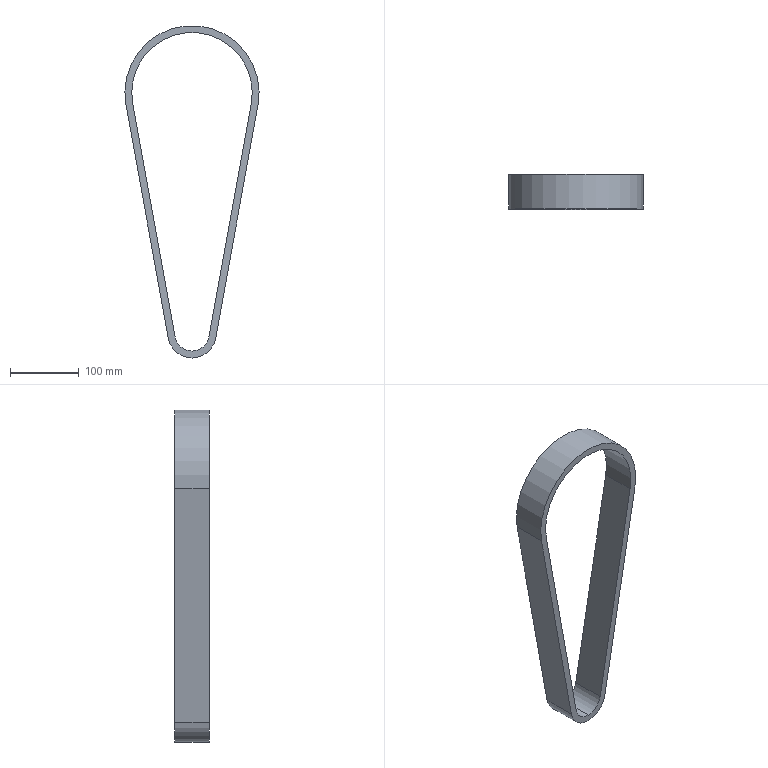Component | SolidWorks | TimingBelt-1 | 1 solid | 12 faces | box 195 x 50 x 482.5 mm | volume 548018 mm3 | cylinder 6 | plane 6 | commonest cylinder face diameters 50 x2 70 x2 195 x1 175 x1 | material Custom Plastic
build123d program:
from build123d import *

# Parameters (mm, degrees)
BOSS_EXTRUDE1_DEPTH = 50


with BuildPart() as part:
    # Sketch1 → Boss-Extrude1 (new body)
    with BuildSketch(Plane.XY):
        with BuildLine():
            Line((-6.25, 34.437), (332.589, 95.933))
            ThreePointArc((332.589, 95.933), (447.5, 0), (332.589, -95.933))
            Line((332.589, -95.933), (-6.25, -34.437))
            ThreePointArc((-6.25, -34.437), (-35, 0), (-6.25, 34.437))
        make_face()
        with BuildLine():
            Line((-4.464, 24.598), (334.375, 86.094))
            ThreePointArc((334.375, 86.094), (437.5, 0), (334.375, -86.094))
            Line((334.375, -86.094), (-4.464, -24.598))
            ThreePointArc((-4.464, -24.598), (-25, 0), (-4.464, 24.598))
        make_face(mode=Mode.SUBTRACT)
    extrude(amount=BOSS_EXTRUDE1_DEPTH)


solid = part.part

# Placed as in the assembly
solid = solid.moved(Location((-371.359, -342.185, 1062), (90, 0, 90)))
STEP:
#1=COLOUR_RGB('',0.7922,0.8196,0.9333);
#2=FILL_AREA_STYLE_COLOUR('',#1);
#3=FILL_AREA_STYLE('',(#2));
#4=SURFACE_STYLE_FILL_AREA(#3);
#5=SURFACE_SIDE_STYLE('',(#4));
#6=SURFACE_STYLE_USAGE(.BOTH.,#5);
#7=PRESENTATION_STYLE_ASSIGNMENT((#6));
#8=CARTESIAN_POINT('',(-13.652,-13.472,41.635));
#9=VERTEX_POINT('',#8);
#10=CARTESIAN_POINT('',(-14.62,-13.472,40.827));
#11=VERTEX_POINT('',#10);
#12=CARTESIAN_POINT('',(-14.62,-13.472,41.811));
#13=DIRECTION('',(0.,1.,0.));
#14=DIRECTION('',(0.,0.,1.));
#15=AXIS2_PLACEMENT_3D('',#12,#13,#14);
#16=CIRCLE('',#15,0.9843);
#17=EDGE_CURVE('',#9,#11,#16,.T.);
#18=ORIENTED_EDGE('',*,*,#17,.T.);
#19=CARTESIAN_POINT('',(-14.62,-15.44,40.827));
#20=VERTEX_POINT('',#19);
#21=CARTESIAN_POINT('',(-14.62,-13.472,40.827));
#22=DIRECTION('',(-0.,-1.,-0.));
#23=VECTOR('',#22,39.37);
#24=LINE('',#21,#23);
#25=EDGE_CURVE('',#11,#20,#24,.T.);
#26=ORIENTED_EDGE('',*,*,#25,.T.);
#27=CARTESIAN_POINT('',(-13.652,-15.44,41.635));
#28=VERTEX_POINT('',#27);
#29=CARTESIAN_POINT('',(-14.62,-15.44,41.811));
#30=DIRECTION('',(0.,1.,0.));
#31=DIRECTION('',(0.,0.,1.));
#32=AXIS2_PLACEMENT_3D('',#29,#30,#31);
#33=CIRCLE('',#32,0.9843);
#34=EDGE_CURVE('',#28,#20,#33,.T.);
#35=ORIENTED_EDGE('',*,*,#34,.F.);
#36=CARTESIAN_POINT('',(-13.652,-13.472,41.635));
#37=DIRECTION('',(-0.,-1.,-0.));
#38=VECTOR('',#37,39.37);
#39=LINE('',#36,#38);
#40=EDGE_CURVE('',#9,#28,#39,.T.);
#41=ORIENTED_EDGE('',*,*,#40,.F.);
#42=EDGE_LOOP('',(#18,#26,#35,#41));
#43=FACE_OUTER_BOUND('',#42,.T.);
#44=CARTESIAN_POINT('',(-14.62,-13.472,41.811));
#45=DIRECTION('',(-0.,-1.,-0.));
#46=DIRECTION('',(0.,0.,-1.));
#47=AXIS2_PLACEMENT_3D('',#44,#45,#46);
#48=CYLINDRICAL_SURFACE('',#47,0.9843);
#49=ADVANCED_FACE('',(#43),#48,.F.);
#50=CARTESIAN_POINT('',(-14.62,-13.472,40.433));
#51=VERTEX_POINT('',#50);
#52=CARTESIAN_POINT('',(-15.976,-13.472,41.565));
#53=VERTEX_POINT('',#52);
#54=CARTESIAN_POINT('',(-14.62,-13.472,41.811));
#55=DIRECTION('',(0.,1.,0.));
#56=DIRECTION('',(0.,0.,1.));
#57=AXIS2_PLACEMENT_3D('',#54,#55,#56);
#58=CIRCLE('',#57,1.378);
#59=EDGE_CURVE('',#51,#53,#58,.T.);
#60=ORIENTED_EDGE('',*,*,#59,.F.);
#61=CARTESIAN_POINT('',(-14.62,-15.44,40.433));
#62=VERTEX_POINT('',#61);
#63=CARTESIAN_POINT('',(-14.62,-13.472,40.433));
#64=DIRECTION('',(-0.,-1.,-0.));
#65=VECTOR('',#64,39.37);
#66=LINE('',#63,#65);
#67=EDGE_CURVE('',#51,#62,#66,.T.);
#68=ORIENTED_EDGE('',*,*,#67,.T.);
#69=CARTESIAN_POINT('',(-15.976,-15.44,41.565));
#70=VERTEX_POINT('',#69);
#71=CARTESIAN_POINT('',(-14.62,-15.44,41.811));
#72=DIRECTION('',(0.,1.,0.));
#73=DIRECTION('',(0.,0.,1.));
#74=AXIS2_PLACEMENT_3D('',#71,#72,#73);
#75=CIRCLE('',#74,1.378);
#76=EDGE_CURVE('',#62,#70,#75,.T.);
#77=ORIENTED_EDGE('',*,*,#76,.T.);
#78=CARTESIAN_POINT('',(-15.976,-13.472,41.565));
#79=DIRECTION('',(-0.,-1.,-0.));
#80=VECTOR('',#79,39.37);
#81=LINE('',#78,#80);
#82=EDGE_CURVE('',#53,#70,#81,.T.);
#83=ORIENTED_EDGE('',*,*,#82,.F.);
#84=EDGE_LOOP('',(#60,#68,#77,#83));
#85=FACE_OUTER_BOUND('',#84,.T.);
#86=CARTESIAN_POINT('',(-14.62,-13.472,41.811));
#87=DIRECTION('',(-0.,-1.,-0.));
#88=DIRECTION('',(0.,0.,-1.));
#89=AXIS2_PLACEMENT_3D('',#86,#87,#88);
#90=CYLINDRICAL_SURFACE('',#89,1.378);
#91=ADVANCED_FACE('',(#85),#90,.T.);
#92=CARTESIAN_POINT('',(-13.265,-13.472,41.565));
#93=VERTEX_POINT('',#92);
#94=CARTESIAN_POINT('',(-14.62,-13.472,41.811));
#95=DIRECTION('',(0.,1.,0.));
#96=DIRECTION('',(0.,0.,1.));
#97=AXIS2_PLACEMENT_3D('',#94,#95,#96);
#98=CIRCLE('',#97,1.378);
#99=EDGE_CURVE('',#93,#51,#98,.T.);
#100=ORIENTED_EDGE('',*,*,#99,.T.);
#101=ORIENTED_EDGE('',*,*,#59,.T.);
#102=CARTESIAN_POINT('',(-18.397,-13.472,54.905));
#103=VERTEX_POINT('',#102);
#104=CARTESIAN_POINT('',(-15.976,-13.472,41.565));
#105=DIRECTION('',(-0.1786,-0.,0.9839));
#106=VECTOR('',#105,39.37);
#107=LINE('',#104,#106);
#108=EDGE_CURVE('',#53,#103,#107,.T.);
#109=ORIENTED_EDGE('',*,*,#108,.T.);
#110=CARTESIAN_POINT('',(-10.844,-13.472,54.905));
#111=VERTEX_POINT('',#110);
#112=CARTESIAN_POINT('',(-14.62,-13.472,55.591));
#113=DIRECTION('',(0.,1.,0.));
#114=DIRECTION('',(0.,0.,1.));
#115=AXIS2_PLACEMENT_3D('',#112,#113,#114);
#116=CIRCLE('',#115,3.839);
#117=EDGE_CURVE('',#103,#111,#116,.T.);
#118=ORIENTED_EDGE('',*,*,#117,.T.);
#119=CARTESIAN_POINT('',(-13.265,-13.472,41.565));
#120=DIRECTION('',(-0.1786,0.,-0.9839));
#121=VECTOR('',#120,39.37);
#122=LINE('',#119,#121);
#123=EDGE_CURVE('',#111,#93,#122,.T.);
#124=ORIENTED_EDGE('',*,*,#123,.T.);
#125=EDGE_LOOP('',(#100,#101,#109,#118,#124));
#126=FACE_OUTER_BOUND('',#125,.T.);
#127=CARTESIAN_POINT('',(-11.231,-13.472,54.975));
#128=VERTEX_POINT('',#127);
#129=CARTESIAN_POINT('',(-13.652,-13.472,41.635));
#130=DIRECTION('',(-0.1786,0.,-0.9839));
#131=VECTOR('',#130,39.37);
#132=LINE('',#129,#131);
#133=EDGE_CURVE('',#128,#9,#132,.T.);
#134=ORIENTED_EDGE('',*,*,#133,.F.);
#135=CARTESIAN_POINT('',(-18.01,-13.472,54.975));
#136=VERTEX_POINT('',#135);
#137=CARTESIAN_POINT('',(-14.62,-13.472,55.591));
#138=DIRECTION('',(0.,1.,0.));
#139=DIRECTION('',(0.,0.,1.));
#140=AXIS2_PLACEMENT_3D('',#137,#138,#139);
#141=CIRCLE('',#140,3.445);
#142=EDGE_CURVE('',#136,#128,#141,.T.);
#143=ORIENTED_EDGE('',*,*,#142,.F.);
#144=CARTESIAN_POINT('',(-15.589,-13.472,41.635));
#145=VERTEX_POINT('',#144);
#146=CARTESIAN_POINT('',(-15.589,-13.472,41.635));
#147=DIRECTION('',(-0.1786,-0.,0.9839));
#148=VECTOR('',#147,39.37);
#149=LINE('',#146,#148);
#150=EDGE_CURVE('',#145,#136,#149,.T.);
#151=ORIENTED_EDGE('',*,*,#150,.F.);
#152=CARTESIAN_POINT('',(-14.62,-13.472,41.811));
#153=DIRECTION('',(0.,1.,0.));
#154=DIRECTION('',(0.,0.,1.));
#155=AXIS2_PLACEMENT_3D('',#152,#153,#154);
#156=CIRCLE('',#155,0.9843);
#157=EDGE_CURVE('',#11,#145,#156,.T.);
#158=ORIENTED_EDGE('',*,*,#157,.F.);
#159=ORIENTED_EDGE('',*,*,#17,.F.);
#160=EDGE_LOOP('',(#134,#143,#151,#158,#159));
#161=FACE_BOUND('',#160,.T.);
#162=CARTESIAN_POINT('',(-14.62,-13.472,41.811));
#163=DIRECTION('',(0.,1.,0.));
#164=DIRECTION('',(-0.,-0.,1.));
#165=AXIS2_PLACEMENT_3D('',#162,#163,#164);
#166=PLANE('',#165);
#167=ADVANCED_FACE('',(#126,#161),#166,.T.);
#168=CARTESIAN_POINT('',(-13.265,-15.44,41.565));
#169=VERTEX_POINT('',#168);
#170=CARTESIAN_POINT('',(-14.62,-15.44,41.811));
#171=DIRECTION('',(0.,1.,0.));
#172=DIRECTION('',(0.,0.,1.));
#173=AXIS2_PLACEMENT_3D('',#170,#171,#172);
#174=CIRCLE('',#173,1.378);
#175=EDGE_CURVE('',#169,#62,#174,.T.);
#176=ORIENTED_EDGE('',*,*,#175,.F.);
#177=CARTESIAN_POINT('',(-10.844,-15.44,54.905));
#178=VERTEX_POINT('',#177);
#179=CARTESIAN_POINT('',(-13.265,-15.44,41.565));
#180=DIRECTION('',(-0.1786,0.,-0.9839));
#181=VECTOR('',#180,39.37);
#182=LINE('',#179,#181);
#183=EDGE_CURVE('',#178,#169,#182,.T.);
#184=ORIENTED_EDGE('',*,*,#183,.F.);
#185=CARTESIAN_POINT('',(-18.397,-15.44,54.905));
#186=VERTEX_POINT('',#185);
#187=CARTESIAN_POINT('',(-14.62,-15.44,55.591));
#188=DIRECTION('',(0.,1.,0.));
#189=DIRECTION('',(0.,0.,1.));
#190=AXIS2_PLACEMENT_3D('',#187,#188,#189);
#191=CIRCLE('',#190,3.839);
#192=EDGE_CURVE('',#186,#178,#191,.T.);
#193=ORIENTED_EDGE('',*,*,#192,.F.);
#194=CARTESIAN_POINT('',(-15.976,-15.44,41.565));
#195=DIRECTION('',(-0.1786,-0.,0.9839));
#196=VECTOR('',#195,39.37);
#197=LINE('',#194,#196);
#198=EDGE_CURVE('',#70,#186,#197,.T.);
#199=ORIENTED_EDGE('',*,*,#198,.F.);
#200=ORIENTED_EDGE('',*,*,#76,.F.);
#201=EDGE_LOOP('',(#176,#184,#193,#199,#200));
#202=FACE_OUTER_BOUND('',#201,.T.);
#203=CARTESIAN_POINT('',(-18.01,-15.44,54.975));
#204=VERTEX_POINT('',#203);
#205=CARTESIAN_POINT('',(-11.231,-15.44,54.975));
#206=VERTEX_POINT('',#205);
#207=CARTESIAN_POINT('',(-14.62,-15.44,55.591));
#208=DIRECTION('',(0.,1.,0.));
#209=DIRECTION('',(0.,0.,1.));
#210=AXIS2_PLACEMENT_3D('',#207,#208,#209);
#211=CIRCLE('',#210,3.445);
#212=EDGE_CURVE('',#204,#206,#211,.T.);
#213=ORIENTED_EDGE('',*,*,#212,.T.);
#214=CARTESIAN_POINT('',(-13.652,-15.44,41.635));
#215=DIRECTION('',(-0.1786,0.,-0.9839));
#216=VECTOR('',#215,39.37);
#217=LINE('',#214,#216);
#218=EDGE_CURVE('',#206,#28,#217,.T.);
#219=ORIENTED_EDGE('',*,*,#218,.T.);
#220=ORIENTED_EDGE('',*,*,#34,.T.);
#221=CARTESIAN_POINT('',(-15.589,-15.44,41.635));
#222=VERTEX_POINT('',#221);
#223=CARTESIAN_POINT('',(-14.62,-15.44,41.811));
#224=DIRECTION('',(0.,1.,0.));
#225=DIRECTION('',(0.,0.,1.));
#226=AXIS2_PLACEMENT_3D('',#223,#224,#225);
#227=CIRCLE('',#226,0.9843);
#228=EDGE_CURVE('',#20,#222,#227,.T.);
#229=ORIENTED_EDGE('',*,*,#228,.T.);
#230=CARTESIAN_POINT('',(-15.589,-15.44,41.635));
#231=DIRECTION('',(-0.1786,-0.,0.9839));
#232=VECTOR('',#231,39.37);
#233=LINE('',#230,#232);
#234=EDGE_CURVE('',#222,#204,#233,.T.);
#235=ORIENTED_EDGE('',*,*,#234,.T.);
#236=EDGE_LOOP('',(#213,#219,#220,#229,#235));
#237=FACE_BOUND('',#236,.T.);
#238=CARTESIAN_POINT('',(-14.62,-15.44,41.811));
#239=DIRECTION('',(0.,1.,0.));
#240=DIRECTION('',(-0.,-0.,1.));
#241=AXIS2_PLACEMENT_3D('',#238,#239,#240);
#242=PLANE('',#241);
#243=ADVANCED_FACE('',(#202,#237),#242,.F.);
#244=ORIENTED_EDGE('',*,*,#67,.F.);
#245=ORIENTED_EDGE('',*,*,#99,.F.);
#246=CARTESIAN_POINT('',(-13.265,-13.472,41.565));
#247=DIRECTION('',(-0.,-1.,-0.));
#248=VECTOR('',#247,39.37);
#249=LINE('',#246,#248);
#250=EDGE_CURVE('',#93,#169,#249,.T.);
#251=ORIENTED_EDGE('',*,*,#250,.T.);
#252=ORIENTED_EDGE('',*,*,#175,.T.);
#253=EDGE_LOOP('',(#244,#245,#251,#252));
#254=FACE_OUTER_BOUND('',#253,.T.);
#255=CARTESIAN_POINT('',(-14.62,-13.472,41.811));
#256=DIRECTION('',(-0.,-1.,-0.));
#257=DIRECTION('',(0.,0.,-1.));
#258=AXIS2_PLACEMENT_3D('',#255,#256,#257);
#259=CYLINDRICAL_SURFACE('',#258,1.378);
#260=ADVANCED_FACE('',(#254),#259,.T.);
#261=ORIENTED_EDGE('',*,*,#198,.T.);
#262=CARTESIAN_POINT('',(-18.397,-13.472,54.905));
#263=DIRECTION('',(-0.,-1.,-0.));
#264=VECTOR('',#263,39.37);
#265=LINE('',#262,#264);
#266=EDGE_CURVE('',#103,#186,#265,.T.);
#267=ORIENTED_EDGE('',*,*,#266,.F.);
#268=ORIENTED_EDGE('',*,*,#108,.F.);
#269=ORIENTED_EDGE('',*,*,#82,.T.);
#270=EDGE_LOOP('',(#261,#267,#268,#269));
#271=FACE_OUTER_BOUND('',#270,.T.);
#272=CARTESIAN_POINT('',(-15.976,-13.472,41.565));
#273=DIRECTION('',(0.9839,-0.,0.1786));
#274=DIRECTION('',(0.1786,0.,-0.9839));
#275=AXIS2_PLACEMENT_3D('',#272,#273,#274);
#276=PLANE('',#275);
#277=ADVANCED_FACE('',(#271),#276,.F.);
#278=ORIENTED_EDGE('',*,*,#192,.T.);
#279=CARTESIAN_POINT('',(-10.844,-13.472,54.905));
#280=DIRECTION('',(-0.,-1.,-0.));
#281=VECTOR('',#280,39.37);
#282=LINE('',#279,#281);
#283=EDGE_CURVE('',#111,#178,#282,.T.);
#284=ORIENTED_EDGE('',*,*,#283,.F.);
#285=ORIENTED_EDGE('',*,*,#117,.F.);
#286=ORIENTED_EDGE('',*,*,#266,.T.);
#287=EDGE_LOOP('',(#278,#284,#285,#286));
#288=FACE_OUTER_BOUND('',#287,.T.);
#289=CARTESIAN_POINT('',(-14.62,-13.472,55.591));
#290=DIRECTION('',(-0.,-1.,-0.));
#291=DIRECTION('',(0.,0.,-1.));
#292=AXIS2_PLACEMENT_3D('',#289,#290,#291);
#293=CYLINDRICAL_SURFACE('',#292,3.839);
#294=ADVANCED_FACE('',(#288),#293,.T.);
#295=ORIENTED_EDGE('',*,*,#183,.T.);
#296=ORIENTED_EDGE('',*,*,#250,.F.);
#297=ORIENTED_EDGE('',*,*,#123,.F.);
#298=ORIENTED_EDGE('',*,*,#283,.T.);
#299=EDGE_LOOP('',(#295,#296,#297,#298));
#300=FACE_OUTER_BOUND('',#299,.T.);
#301=CARTESIAN_POINT('',(-13.265,-13.472,41.565));
#302=DIRECTION('',(-0.9839,0.,0.1786));
#303=DIRECTION('',(0.1786,-0.,0.9839));
#304=AXIS2_PLACEMENT_3D('',#301,#302,#303);
#305=PLANE('',#304);
#306=ADVANCED_FACE('',(#300),#305,.F.);
#307=ORIENTED_EDGE('',*,*,#212,.F.);
#308=CARTESIAN_POINT('',(-18.01,-13.472,54.975));
#309=DIRECTION('',(-0.,-1.,-0.));
#310=VECTOR('',#309,39.37);
#311=LINE('',#308,#310);
#312=EDGE_CURVE('',#136,#204,#311,.T.);
#313=ORIENTED_EDGE('',*,*,#312,.F.);
#314=ORIENTED_EDGE('',*,*,#142,.T.);
#315=CARTESIAN_POINT('',(-11.231,-13.472,54.975));
#316=DIRECTION('',(-0.,-1.,-0.));
#317=VECTOR('',#316,39.37);
#318=LINE('',#315,#317);
#319=EDGE_CURVE('',#128,#206,#318,.T.);
#320=ORIENTED_EDGE('',*,*,#319,.T.);
#321=EDGE_LOOP('',(#307,#313,#314,#320));
#322=FACE_OUTER_BOUND('',#321,.T.);
#323=CARTESIAN_POINT('',(-14.62,-13.472,55.591));
#324=DIRECTION('',(-0.,-1.,-0.));
#325=DIRECTION('',(0.,0.,-1.));
#326=AXIS2_PLACEMENT_3D('',#323,#324,#325);
#327=CYLINDRICAL_SURFACE('',#326,3.445);
#328=ADVANCED_FACE('',(#322),#327,.F.);
#329=ORIENTED_EDGE('',*,*,#218,.F.);
#330=ORIENTED_EDGE('',*,*,#319,.F.);
#331=ORIENTED_EDGE('',*,*,#133,.T.);
#332=ORIENTED_EDGE('',*,*,#40,.T.);
#333=EDGE_LOOP('',(#329,#330,#331,#332));
#334=FACE_OUTER_BOUND('',#333,.T.);
#335=CARTESIAN_POINT('',(-13.652,-13.472,41.635));
#336=DIRECTION('',(-0.9839,0.,0.1786));
#337=DIRECTION('',(0.1786,-0.,0.9839));
#338=AXIS2_PLACEMENT_3D('',#335,#336,#337);
#339=PLANE('',#338);
#340=ADVANCED_FACE('',(#334),#339,.T.);
#341=ORIENTED_EDGE('',*,*,#25,.F.);
#342=ORIENTED_EDGE('',*,*,#157,.T.);
#343=CARTESIAN_POINT('',(-15.589,-13.472,41.635));
#344=DIRECTION('',(-0.,-1.,-0.));
#345=VECTOR('',#344,39.37);
#346=LINE('',#343,#345);
#347=EDGE_CURVE('',#145,#222,#346,.T.);
#348=ORIENTED_EDGE('',*,*,#347,.T.);
#349=ORIENTED_EDGE('',*,*,#228,.F.);
#350=EDGE_LOOP('',(#341,#342,#348,#349));
#351=FACE_OUTER_BOUND('',#350,.T.);
#352=CARTESIAN_POINT('',(-14.62,-13.472,41.811));
#353=DIRECTION('',(-0.,-1.,-0.));
#354=DIRECTION('',(0.,0.,-1.));
#355=AXIS2_PLACEMENT_3D('',#352,#353,#354);
#356=CYLINDRICAL_SURFACE('',#355,0.9843);
#357=ADVANCED_FACE('',(#351),#356,.F.);
#358=ORIENTED_EDGE('',*,*,#234,.F.);
#359=ORIENTED_EDGE('',*,*,#347,.F.);
#360=ORIENTED_EDGE('',*,*,#150,.T.);
#361=ORIENTED_EDGE('',*,*,#312,.T.);
#362=EDGE_LOOP('',(#358,#359,#360,#361));
#363=FACE_OUTER_BOUND('',#362,.T.);
#364=CARTESIAN_POINT('',(-15.589,-13.472,41.635));
#365=DIRECTION('',(0.9839,-0.,0.1786));
#366=DIRECTION('',(0.1786,0.,-0.9839));
#367=AXIS2_PLACEMENT_3D('',#364,#365,#366);
#368=PLANE('',#367);
#369=ADVANCED_FACE('',(#363),#368,.T.);
#370=CLOSED_SHELL('',(#49,#91,#167,#243,#260,#277,#294,#306,#328,#340,#357,#369));
#371=MANIFOLD_SOLID_BREP('',#370);
#372=STYLED_ITEM('',(#7),#371);
#373=PRESENTATION_LAYER_ASSIGNMENT('','',(#372));
#374=(LENGTH_UNIT()NAMED_UNIT(*)SI_UNIT($,.METRE.));
#375=LENGTH_MEASURE_WITH_UNIT(LENGTH_MEASURE(0.0254),#374);
#376=DIMENSIONAL_EXPONENTS(1.,0.,0.,0.,0.,0.,0.);
#377=(CONVERSION_BASED_UNIT('',#375)LENGTH_UNIT()NAMED_UNIT(#376));
#378=UNCERTAINTY_MEASURE_WITH_UNIT(LENGTH_MEASURE(0.00001),#377,'','');
#379=(NAMED_UNIT(*)PLANE_ANGLE_UNIT()SI_UNIT($,.RADIAN.));
#380=(NAMED_UNIT(*)SI_UNIT($,.STERADIAN.)SOLID_ANGLE_UNIT());
#381=(GEOMETRIC_REPRESENTATION_CONTEXT(3)GLOBAL_UNCERTAINTY_ASSIGNED_CONTEXT((#378))GLOBAL_UNIT_ASSIGNED_CONTEXT((#377,#379,#380))REPRESENTATION_CONTEXT('',''));
#382=MECHANICAL_DESIGN_GEOMETRIC_PRESENTATION_REPRESENTATION('',(#372),#381);
#383=CARTESIAN_POINT('',(0.,0.,0.));
#384=DIRECTION('',(0.,0.,1.));
#385=DIRECTION('',(1.,0.,0.));
#386=AXIS2_PLACEMENT_3D('',#383,#384,#385);
#387=(LENGTH_UNIT()NAMED_UNIT(*)SI_UNIT($,.METRE.));
#388=LENGTH_MEASURE_WITH_UNIT(LENGTH_MEASURE(0.0254),#387);
#389=DIMENSIONAL_EXPONENTS(1.,0.,0.,0.,0.,0.,0.);
#390=(CONVERSION_BASED_UNIT('',#388)LENGTH_UNIT()NAMED_UNIT(#389));
#391=UNCERTAINTY_MEASURE_WITH_UNIT(LENGTH_MEASURE(0.00001),#390,'','');
#392=(NAMED_UNIT(*)PLANE_ANGLE_UNIT()SI_UNIT($,.RADIAN.));
#393=(NAMED_UNIT(*)SI_UNIT($,.STERADIAN.)SOLID_ANGLE_UNIT());
#394=(GEOMETRIC_REPRESENTATION_CONTEXT(3)GLOBAL_UNCERTAINTY_ASSIGNED_CONTEXT((#391))GLOBAL_UNIT_ASSIGNED_CONTEXT((#390,#392,#393))REPRESENTATION_CONTEXT('',''));
#395=ADVANCED_BREP_SHAPE_REPRESENTATION('',(#371,#386),#394);